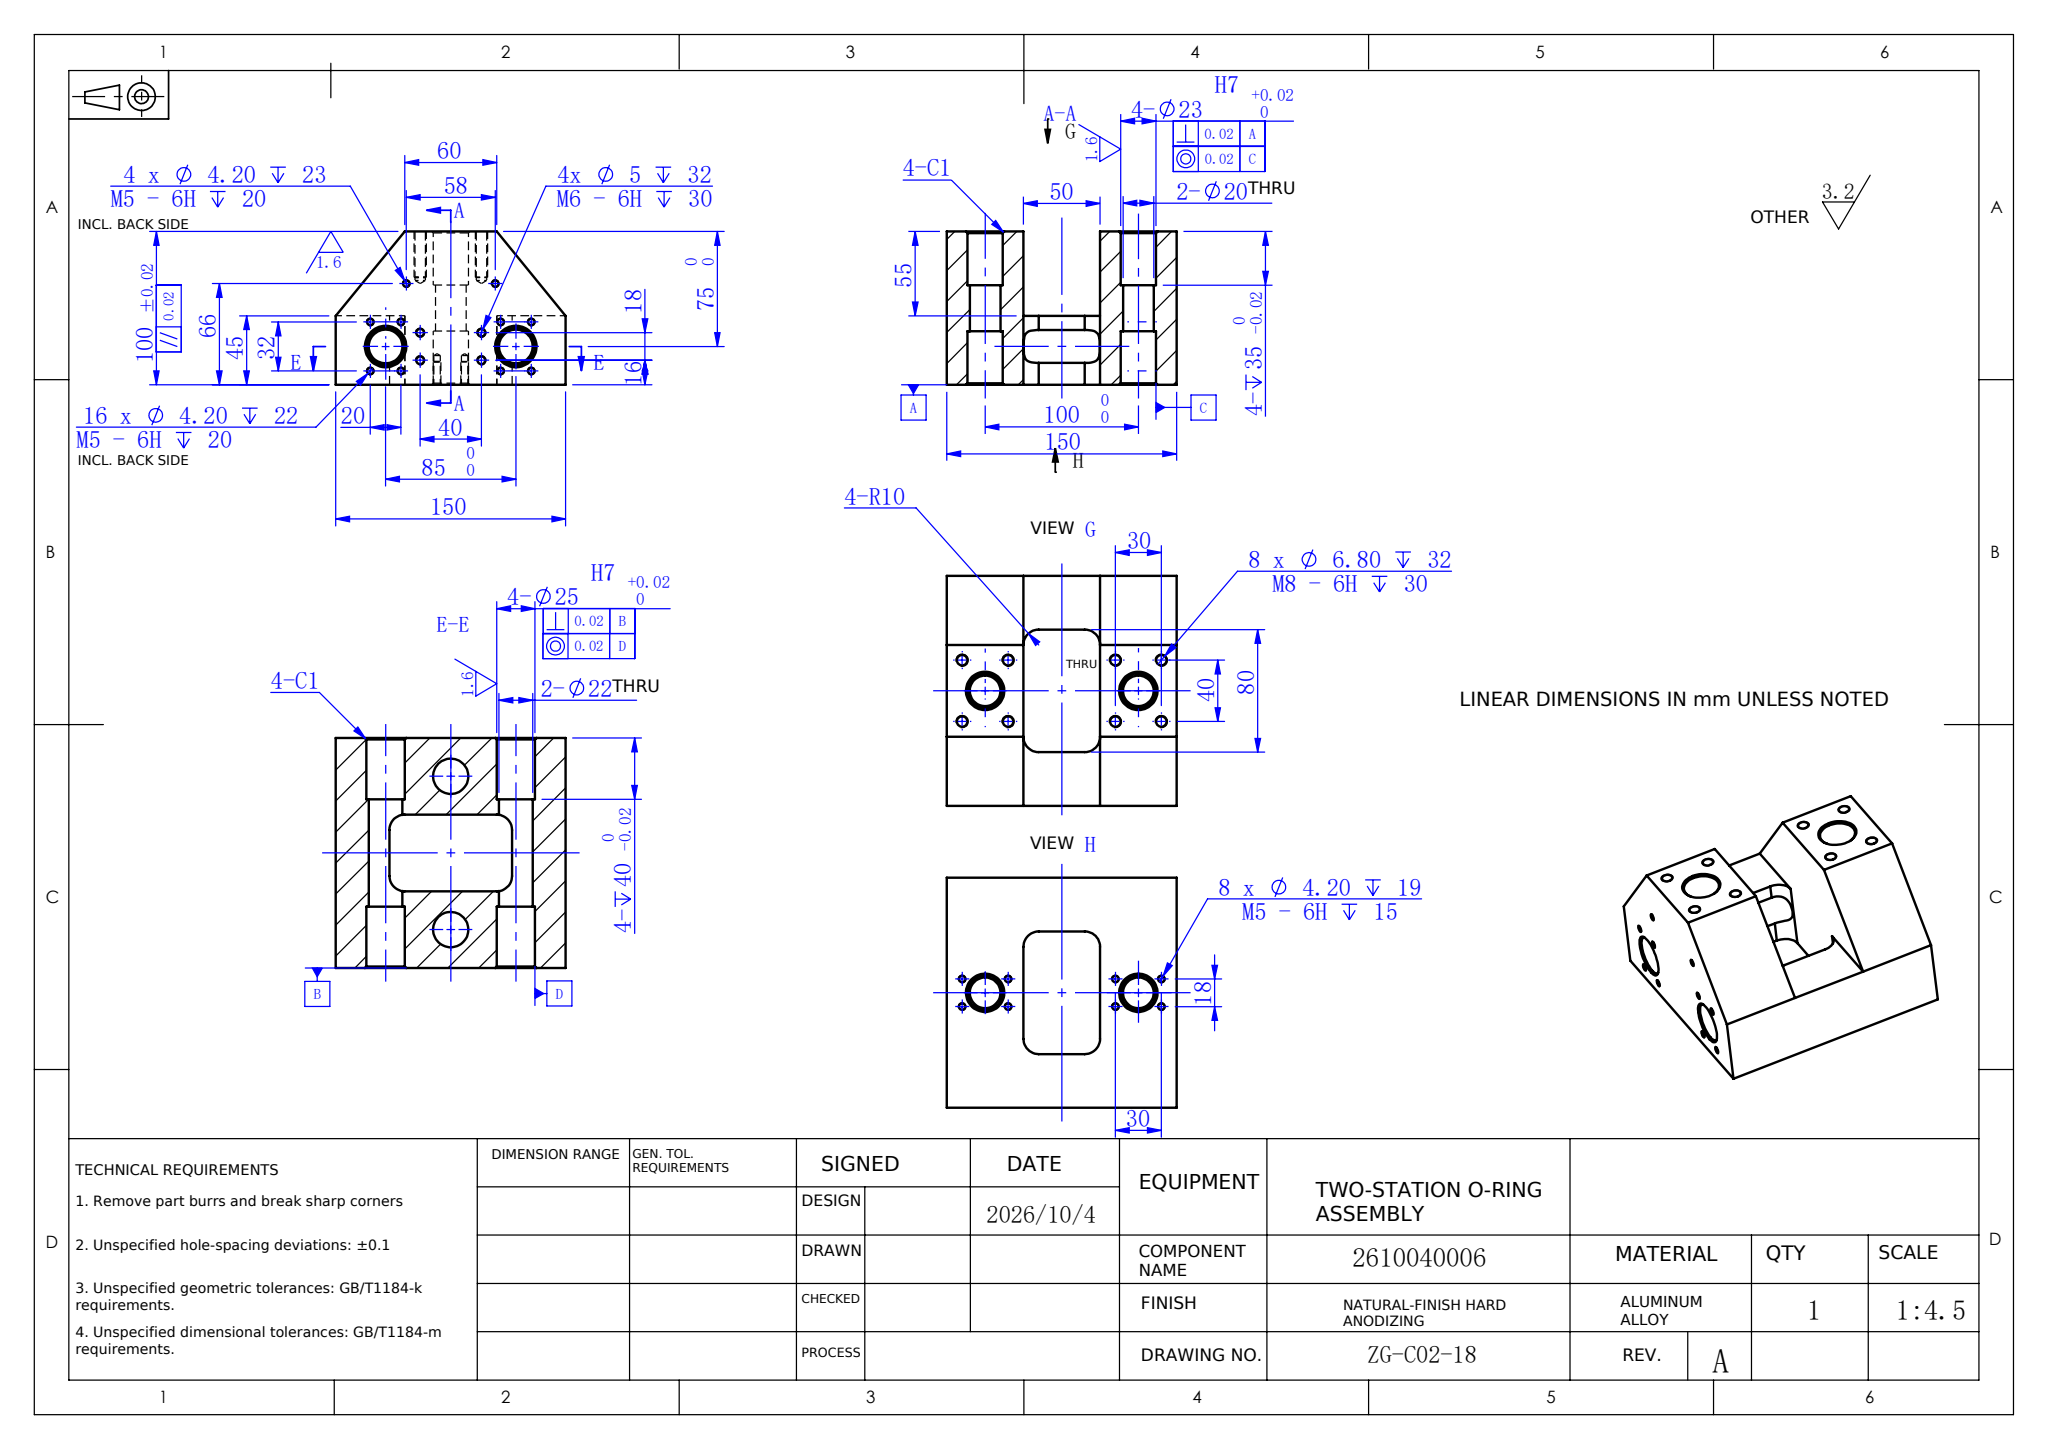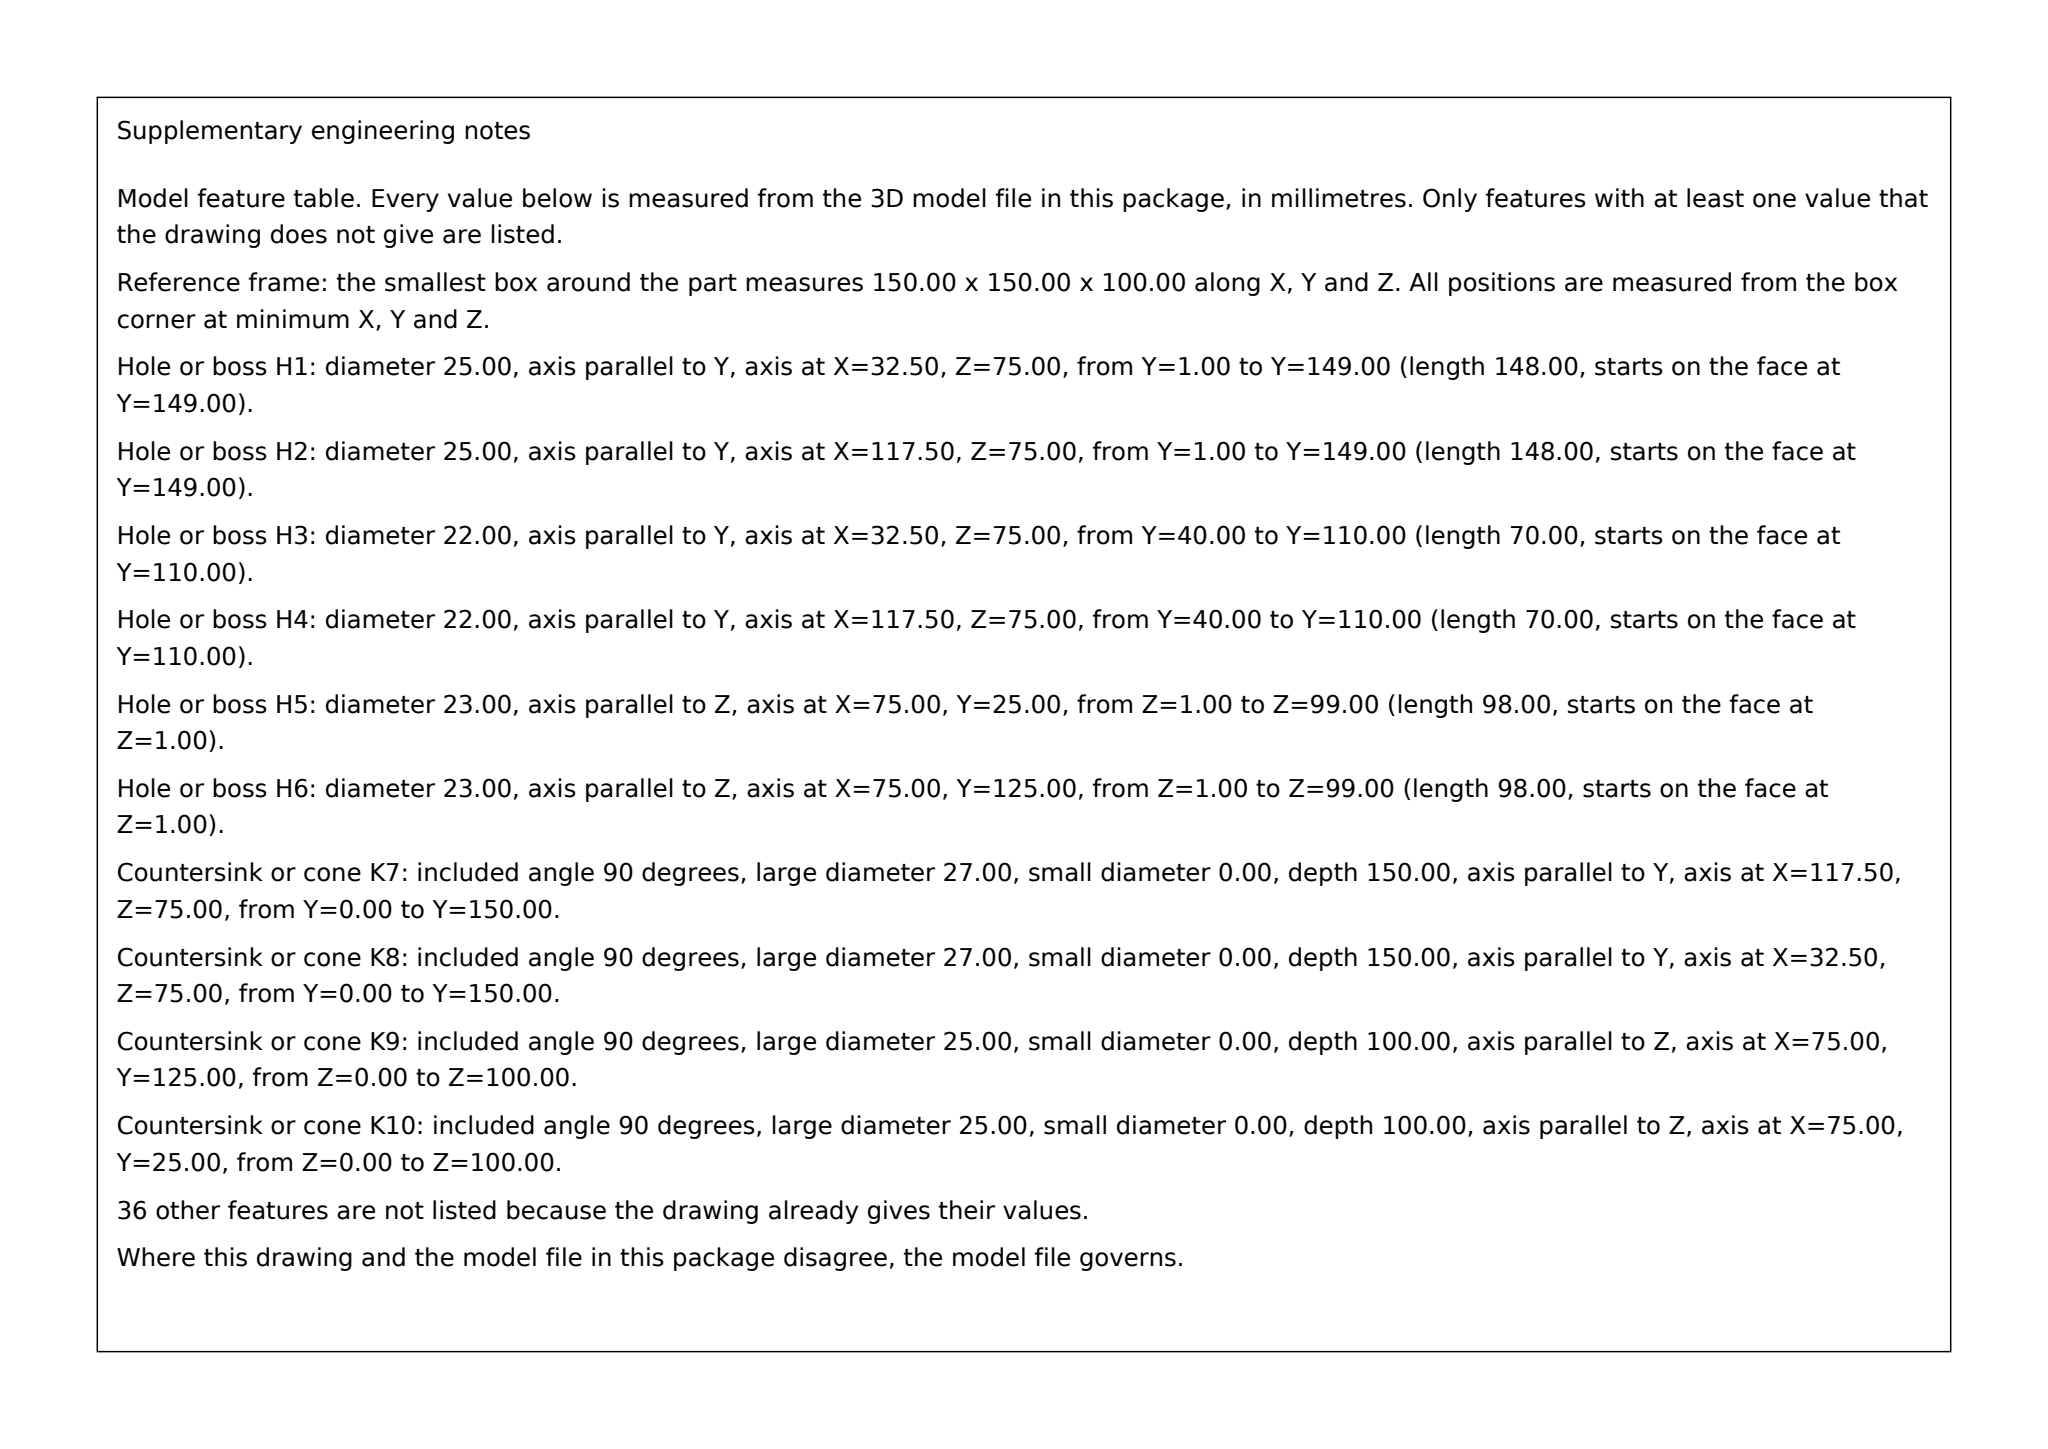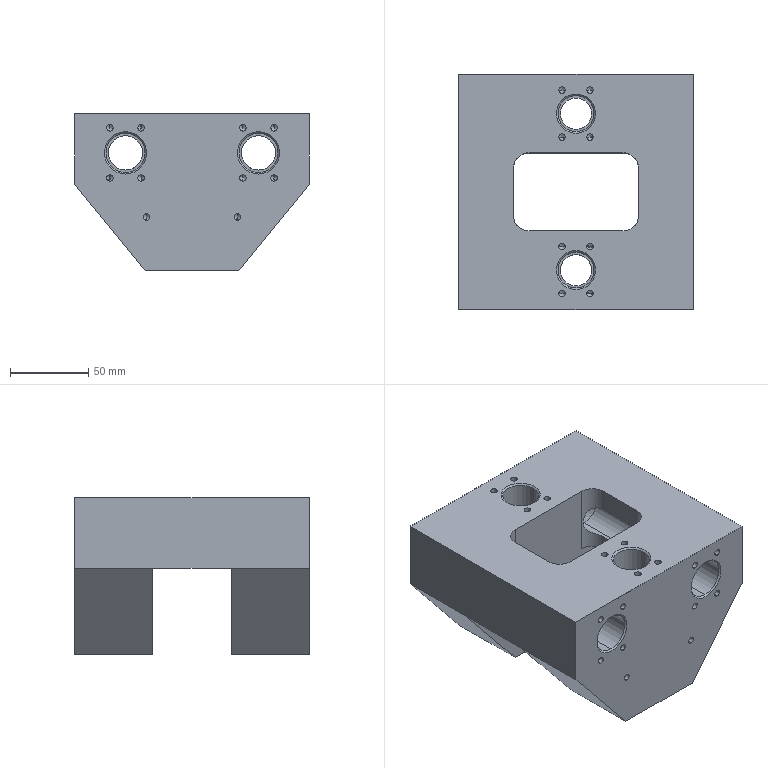Part | SolidWorks | mm | material ALUMINUM ALLOY | 1 solid | 231 faces | box 150 x 150 x 100 mm | volume 1196207 mm3 | cylinder 108 | cone 96 | plane 27 | commonest cylinder face diameters 4.2 x56 6.8 x16 5 x8 25 x8 20 x8 23 x8 22 x4
build123d program:
from build123d import *

# Parameters (mm, degrees)
SKETCH1_W                  = 150
SKETCH1_H                  = 150
BOSS_EXTRUDE1_DEPTH        = 100
SKETCH2_W                  = 80
SKETCH2_H                  = 50
CUT_EXTRUDE1_DEPTH         = 165.663
FILLET1_R                  = 10
SKETCH3_W                  = 55
SKETCH3_H                  = 50
CUT_EXTRUDE2_DEPTH         = 200.776
SKETCH4_R                  = 11.5
CUT_EXTRUDE3_DEPTH         = 35
CUT_EXTRUDE4_START         = -35
SKETCH5_R                  = 11.5
CUT_EXTRUDE4_DEPTH         = 35
SKETCH6_R                  = 10
CUT_EXTRUDE5_DEPTH         = 147.079
CHAMFER1_SIZE              = 1
CUT_EXTRUDE6_DEPTH         = 206.435
M8_TAPPED_HOLE1_D          = 6.8
M8_TAPPED_HOLE1_DEPTH      = 32
M8_TAPPED_HOLE1_TIP        = 2.043
SKETCH10_R                 = 12.5
CUT_EXTRUDE7_DEPTH         = 40
SKETCH13_R                 = 11
CUT_EXTRUDE12_DEPTH        = 179.335
CUT_EXTRUDE13_START        = -40
SKETCH14_R                 = 12.5
CUT_EXTRUDE13_DEPTH        = 40
CHAMFER2_SIZE              = 1
M5_TAPPED_HOLE1_AT_2_COUNT = 2
M5_TAPPED_HOLE1_AT_2_PITCH = 32
M5_TAPPED_HOLE1_AT_3_COUNT = 2
M5_TAPPED_HOLE1_AT_3_PITCH = 37.736
M5_TAPPED_HOLE1_AT_4_COUNT = 2
M5_TAPPED_HOLE1_AT_4_PITCH = 20
M5_TAPPED_HOLE1_AT_5_COUNT = 2
M5_TAPPED_HOLE1_AT_5_PITCH = 85
M5_TAPPED_HOLE1_AT_6_COUNT = 2
M5_TAPPED_HOLE1_AT_6_PITCH = 105
M5_TAPPED_HOLE1_AT_7_COUNT = 2
M5_TAPPED_HOLE1_AT_7_PITCH = 90.824
M5_TAPPED_HOLE1_AT_8_COUNT = 2
M5_TAPPED_HOLE1_AT_8_PITCH = 109.768
M6_TAPPED_HOLE1_D          = 5
M6_TAPPED_HOLE1_DEPTH      = 32
M6_TAPPED_HOLE1_TIP        = 1.502
M5_TAPPED_HOLE2_AT_2_COUNT = 2
M5_TAPPED_HOLE2_AT_2_PITCH = 58
M5_TAPPED_HOLE3_D          = 4.2
M5_TAPPED_HOLE3_DEPTH      = 19
M5_TAPPED_HOLE3_TIP        = 1.262


with BuildPart() as part:
    # Sketch1 → Boss-Extrude1 (new body)
    with BuildSketch(Plane.XY):
        with Locations((-23.506, 11.084)):
            Rectangle(SKETCH1_W, SKETCH1_H)
    extrude(amount=BOSS_EXTRUDE1_DEPTH)

    # Sketch2 → Cut-Extrude1 (cut, through all)
    with BuildSketch(Plane.XY.offset(100)):
        with Locations((-23.506, 11.084)):
            Rectangle(SKETCH2_W, SKETCH2_H)
    extrude(amount=-CUT_EXTRUDE1_DEPTH, mode=Mode.SUBTRACT)

    # Fillet1
    fillet1_edges = [part.edges().sort_by_distance(p)[0] for p in [
        (-63.506, -13.916, 50),
        (-63.506, 36.084, 50),
        (16.494, 36.084, 50),
        (16.494, -13.916, 50),
    ]]
    fillet(fillet1_edges, radius=FILLET1_R)

    # Sketch3 → Cut-Extrude2 (cut, through all)
    with BuildSketch(Plane(origin=(51.494, 0, 0), x_dir=(0, 0, -1), z_dir=(1, 0, 0))):
        with Locations((-27.5, 11.084)):
            Rectangle(SKETCH3_W, SKETCH3_H)
    extrude(amount=-CUT_EXTRUDE2_DEPTH, mode=Mode.SUBTRACT)

    # Sketch4 → Cut-Extrude3 (cut)
    with BuildSketch(Plane(origin=(0, 0, 0), x_dir=(-1, 0, 0), z_dir=(0, 0, -1))):
        with Locations((23.506, -38.916)):
            Circle(SKETCH4_R)
        with Locations((23.506, 61.084)):
            Circle(SKETCH4_R)
    extrude(amount=-CUT_EXTRUDE3_DEPTH, mode=Mode.SUBTRACT)

    # Sketch5 → Cut-Extrude4 (cut)
    with BuildSketch(Plane.XY.offset(100).offset(CUT_EXTRUDE4_START)):
        with Locations(Location((-23.506, 61.084, 0), (0, 0, 180))):
            Circle(SKETCH5_R)
        with Locations(Location((-23.506, -38.916, 0), (0, 0, 180))):
            Circle(SKETCH5_R)
    extrude(amount=CUT_EXTRUDE4_DEPTH, mode=Mode.SUBTRACT)

    # Sketch6 → Cut-Extrude5 (cut, through all)
    with BuildSketch(Plane.XY.offset(65)):
        with Locations((-23.506, 61.084)):
            Circle(SKETCH6_R)
        with Locations((-23.506, -38.916)):
            Circle(SKETCH6_R)
    extrude(amount=-CUT_EXTRUDE5_DEPTH, mode=Mode.SUBTRACT)

    # Chamfer1
    chamfer1_edges = [part.edges().sort_by_distance(p)[0] for p in [
        (-12.006, -38.916, 100),
        (-12.006, -38.916, 0),
        (-12.006, 61.084, 0),
        (-12.006, 61.084, 100),
    ]]
    chamfer(chamfer1_edges, length=CHAMFER1_SIZE)

    # Sketch7 → Cut-Extrude6 (cut, through all)
    with BuildSketch(Plane(origin=(0, -63.916, 0), x_dir=(-1, 0, 0), z_dir=(0, -1, 0))):
        Polygon((53.506, 0), (98.506, -55), (98.506, 0), align=None)
        Polygon((-51.494, 0), (-51.494, -55), (-6.494, 0), align=None)
    extrude(amount=-CUT_EXTRUDE6_DEPTH, mode=Mode.SUBTRACT)

    # M8 Tapped Hole1
    with Locations(Plane(origin=(0, 0, 0), x_dir=(-1, 0, 0), z_dir=(0, 0, -1))):
        with Locations((43.506, -53.916), (43.506, -23.916), (3.506, -23.916), (3.506, -53.916), (3.506, 46.084), (3.506, 76.084), (43.506, 76.084), (43.506, 46.084)):
            Hole(M8_TAPPED_HOLE1_D / 2, depth=M8_TAPPED_HOLE1_DEPTH)
            with Locations((0, 0, -(M8_TAPPED_HOLE1_DEPTH + M8_TAPPED_HOLE1_TIP / 2))):  # 118° drill point
                Cone(0, M8_TAPPED_HOLE1_D / 2, M8_TAPPED_HOLE1_TIP, mode=Mode.SUBTRACT)

    # Sketch10 → Cut-Extrude7 (cut)
    with BuildSketch(Plane(origin=(0, 86.084, 0), x_dir=(1, 0, 0), z_dir=(0, 1, 0))):
        with Locations(Location((-66.006, -75, 0), (0, 0, 270))):
            Circle(SKETCH10_R)
        with Locations(Location((18.994, -75, 0), (0, 0, 270))):
            Circle(SKETCH10_R)
    extrude(amount=-CUT_EXTRUDE7_DEPTH, mode=Mode.SUBTRACT)

    # Sketch13 → Cut-Extrude12 (cut, through all)
    with BuildSketch(Plane(origin=(0, 46.084, 0), x_dir=(1, 0, 0), z_dir=(0, 1, 0))):
        with Locations(Location((-66.006, -75, 0), (0, 0, 270))):
            Circle(SKETCH13_R)
        with Locations(Location((18.994, -75, 0), (0, 0, 270))):
            Circle(SKETCH13_R)
    extrude(amount=-CUT_EXTRUDE12_DEPTH, mode=Mode.SUBTRACT)

    # Sketch14 → Cut-Extrude13 (cut)
    with BuildSketch(Plane(origin=(0, -63.916, 0), x_dir=(-1, 0, 0), z_dir=(0, -1, 0)).offset(CUT_EXTRUDE13_START)):
        with Locations(Location((-18.994, -75, 0), (0, 0, 270))):
            Circle(SKETCH14_R)
        with Locations(Location((66.006, -75, 0), (0, 0, 270))):
            Circle(SKETCH14_R)
    extrude(amount=CUT_EXTRUDE13_DEPTH, mode=Mode.SUBTRACT)

    # Chamfer2
    chamfer2_edges = [part.edges().sort_by_distance(p)[0] for p in [
        (-66.006, 86.084, 62.5),
        (18.994, 86.084, 62.5),
        (18.994, -63.916, 62.5),
        (-66.006, -63.916, 62.5),
    ]]
    chamfer(chamfer2_edges, length=CHAMFER2_SIZE)

    # Sketch15 → M5 Tapped Hole1 (revolve, cut)
    with BuildSketch(Plane(origin=(28.994, -63.916, 91), x_dir=(0, 0, -1), z_dir=(1, 0, 0))):
        Polygon((0, 0), (0, 23.262), (2.1, 22), (2.1, 0), align=None)
    m5_tapped_hole1 = revolve(axis=Axis((28.994, -70.266, 91), (0, 1, 0)), mode=Mode.SUBTRACT)

    # M5 Tapped Hole1 at 2: M5 Tapped Hole1 ×2
    with Locations(*[(0, 0, -i * M5_TAPPED_HOLE1_AT_2_PITCH) for i in range(1, M5_TAPPED_HOLE1_AT_2_COUNT)]):
        add(m5_tapped_hole1, mode=Mode.SUBTRACT)

    # M5 Tapped Hole1 at 3: M5 Tapped Hole1 ×2
    with Locations(*[Vector(-0.53, 0, -0.848) * (i * M5_TAPPED_HOLE1_AT_3_PITCH) for i in range(1, M5_TAPPED_HOLE1_AT_3_COUNT)]):
        add(m5_tapped_hole1, mode=Mode.SUBTRACT)

    # M5 Tapped Hole1 at 4: M5 Tapped Hole1 ×2
    with Locations(*[(-i * M5_TAPPED_HOLE1_AT_4_PITCH, 0, 0) for i in range(1, M5_TAPPED_HOLE1_AT_4_COUNT)]):
        add(m5_tapped_hole1, mode=Mode.SUBTRACT)

    # M5 Tapped Hole1 at 5: M5 Tapped Hole1 ×2
    with Locations(*[(-i * M5_TAPPED_HOLE1_AT_5_PITCH, 0, 0) for i in range(1, M5_TAPPED_HOLE1_AT_5_COUNT)]):
        add(m5_tapped_hole1, mode=Mode.SUBTRACT)

    # M5 Tapped Hole1 at 6: M5 Tapped Hole1 ×2
    with Locations(*[(-i * M5_TAPPED_HOLE1_AT_6_PITCH, 0, 0) for i in range(1, M5_TAPPED_HOLE1_AT_6_COUNT)]):
        add(m5_tapped_hole1, mode=Mode.SUBTRACT)

    # M5 Tapped Hole1 at 7: M5 Tapped Hole1 ×2
    with Locations(*[Vector(-0.9359, 0, -0.3523) * (i * M5_TAPPED_HOLE1_AT_7_PITCH) for i in range(1, M5_TAPPED_HOLE1_AT_7_COUNT)]):
        add(m5_tapped_hole1, mode=Mode.SUBTRACT)

    # M5 Tapped Hole1 at 8: M5 Tapped Hole1 ×2
    with Locations(*[Vector(-0.9566, 0, -0.2915) * (i * M5_TAPPED_HOLE1_AT_8_PITCH) for i in range(1, M5_TAPPED_HOLE1_AT_8_COUNT)]):
        add(m5_tapped_hole1, mode=Mode.SUBTRACT)

    # Mirror1: M5 Tapped Hole1 across plane
    add(m5_tapped_hole1.mirror(Plane(origin=(0, 11.084, 0), x_dir=(0, 0, 1), z_dir=(0, -1, 0))), mode=Mode.SUBTRACT)

    # Mirror1 copy 1 sketch → Mirror1 copy 1 (revolve, cut)
    with BuildSketch(Plane(origin=(28.994, 86.084, 59), x_dir=(0, 0, -1), z_dir=(1, 0, 0))):
        Polygon((0, 0), (0, -23.262), (2.1, -22), (2.1, 0), align=None)
    revolve(axis=Axis((28.994, 92.434, 59), (0, 1, 0)), mode=Mode.SUBTRACT)

    # Mirror1 copy 2 sketch → Mirror1 copy 2 (revolve, cut)
    with BuildSketch(Plane(origin=(8.994, 86.084, 59), x_dir=(0, 0, -1), z_dir=(1, 0, 0))):
        Polygon((0, 0), (0, -23.262), (2.1, -22), (2.1, 0), align=None)
    revolve(axis=Axis((8.994, 92.434, 59), (0, 1, 0)), mode=Mode.SUBTRACT)

    # Mirror1 copy 3 sketch → Mirror1 copy 3 (revolve, cut)
    with BuildSketch(Plane(origin=(8.994, 86.084, 91), x_dir=(0, 0, -1), z_dir=(1, 0, 0))):
        Polygon((0, 0), (0, -23.262), (2.1, -22), (2.1, 0), align=None)
    revolve(axis=Axis((8.994, 92.434, 91), (0, 1, 0)), mode=Mode.SUBTRACT)

    # Mirror1 copy 4 sketch → Mirror1 copy 4 (revolve, cut)
    with BuildSketch(Plane(origin=(-56.006, 86.084, 91), x_dir=(0, 0, -1), z_dir=(1, 0, 0))):
        Polygon((0, 0), (0, -23.262), (2.1, -22), (2.1, 0), align=None)
    revolve(axis=Axis((-56.006, 92.434, 91), (0, 1, 0)), mode=Mode.SUBTRACT)

    # Mirror1 copy 5 sketch → Mirror1 copy 5 (revolve, cut)
    with BuildSketch(Plane(origin=(-76.006, 86.084, 91), x_dir=(0, 0, -1), z_dir=(1, 0, 0))):
        Polygon((0, 0), (0, -23.262), (2.1, -22), (2.1, 0), align=None)
    revolve(axis=Axis((-76.006, 92.434, 91), (0, 1, 0)), mode=Mode.SUBTRACT)

    # Mirror1 copy 6 sketch → Mirror1 copy 6 (revolve, cut)
    with BuildSketch(Plane(origin=(-56.006, 86.084, 59), x_dir=(0, 0, -1), z_dir=(1, 0, 0))):
        Polygon((0, 0), (0, -23.262), (2.1, -22), (2.1, 0), align=None)
    revolve(axis=Axis((-56.006, 92.434, 59), (0, 1, 0)), mode=Mode.SUBTRACT)

    # Mirror1 copy 7 sketch → Mirror1 copy 7 (revolve, cut)
    with BuildSketch(Plane(origin=(-76.006, 86.084, 59), x_dir=(0, 0, -1), z_dir=(1, 0, 0))):
        Polygon((0, 0), (0, -23.262), (2.1, -22), (2.1, 0), align=None)
    revolve(axis=Axis((-76.006, 92.434, 59), (0, 1, 0)), mode=Mode.SUBTRACT)

    # M6 Tapped Hole1
    with Locations(Plane(origin=(0, 86.084, 0), x_dir=(1, 0, 0), z_dir=(0, 1, 0))):
        with Locations((-43.506, -66), (-3.506, -66), (-3.506, -84), (-43.506, -84)):
            Hole(M6_TAPPED_HOLE1_D / 2, depth=M6_TAPPED_HOLE1_DEPTH)
            with Locations((0, 0, -(M6_TAPPED_HOLE1_DEPTH + M6_TAPPED_HOLE1_TIP / 2))):  # 118° drill point
                Cone(0, M6_TAPPED_HOLE1_D / 2, M6_TAPPED_HOLE1_TIP, mode=Mode.SUBTRACT)

    # Sketch22 → M5 Tapped Hole2 (revolve, cut)
    with BuildSketch(Plane(origin=(-52.506, 86.084, 34), x_dir=(0, 0, 1), z_dir=(1, 0, 0))):
        Polygon((0, 0), (0, 24.262), (2.1, 23), (2.1, 0), align=None)
    m5_tapped_hole2 = revolve(axis=Axis((-52.506, 92.434, 34), (0, -1, 0)), mode=Mode.SUBTRACT)

    # M5 Tapped Hole2 at 2: M5 Tapped Hole2 ×2
    with Locations(*[(i * M5_TAPPED_HOLE2_AT_2_PITCH, 0, 0) for i in range(1, M5_TAPPED_HOLE2_AT_2_COUNT)]):
        add(m5_tapped_hole2, mode=Mode.SUBTRACT)

    # Mirror2: M5 Tapped Hole2 across plane
    add(m5_tapped_hole2.mirror(Plane(origin=(0, 11.084, 0), x_dir=(0, 0, 1), z_dir=(0, -1, 0))), mode=Mode.SUBTRACT)

    # Mirror2 copy 1 sketch → Mirror2 copy 1 (revolve, cut)
    with BuildSketch(Plane(origin=(5.494, -63.916, 34), x_dir=(0, 0, 1), z_dir=(1, 0, 0))):
        Polygon((0, 0), (0, -24.262), (2.1, -23), (2.1, 0), align=None)
    revolve(axis=Axis((5.494, -70.266, 34), (0, -1, 0)), mode=Mode.SUBTRACT)

    # M5 Tapped Hole3
    with Locations(Plane.XY.offset(100)):
        with Locations((-32.506, -53.916), (-32.506, -23.916), (-14.506, -23.916), (-14.506, -53.916), (-32.506, 46.084), (-32.506, 76.084), (-14.506, 76.084), (-14.506, 46.084)):
            Hole(M5_TAPPED_HOLE3_D / 2, depth=M5_TAPPED_HOLE3_DEPTH)
            with Locations((0, 0, -(M5_TAPPED_HOLE3_DEPTH + M5_TAPPED_HOLE3_TIP / 2))):  # 118° drill point
                Cone(0, M5_TAPPED_HOLE3_D / 2, M5_TAPPED_HOLE3_TIP, mode=Mode.SUBTRACT)


solid = part.part